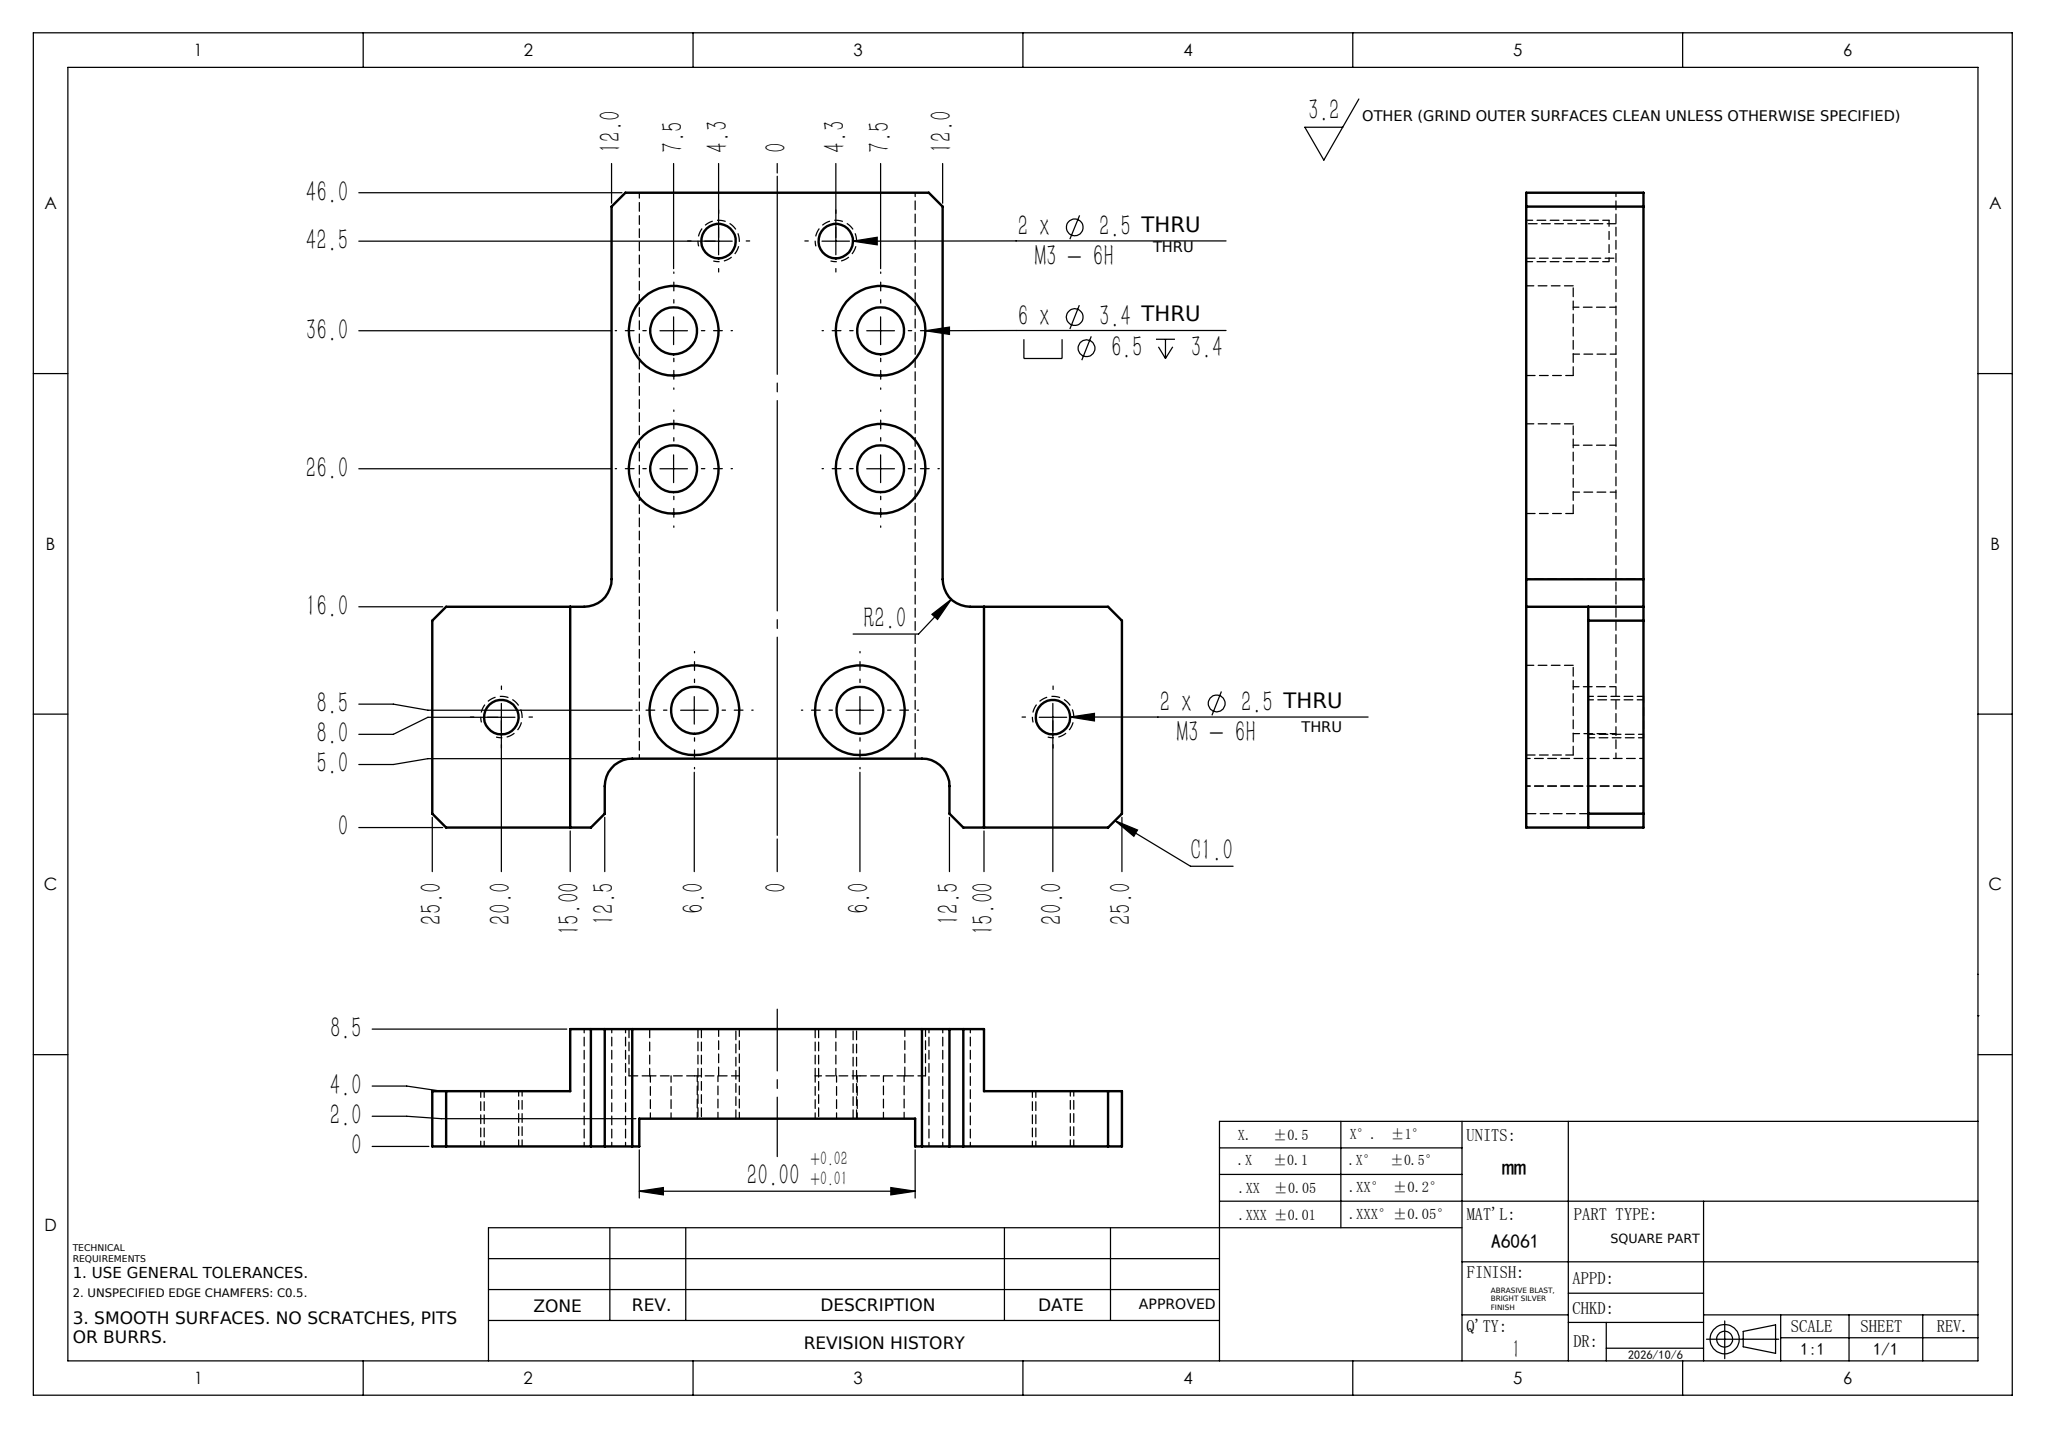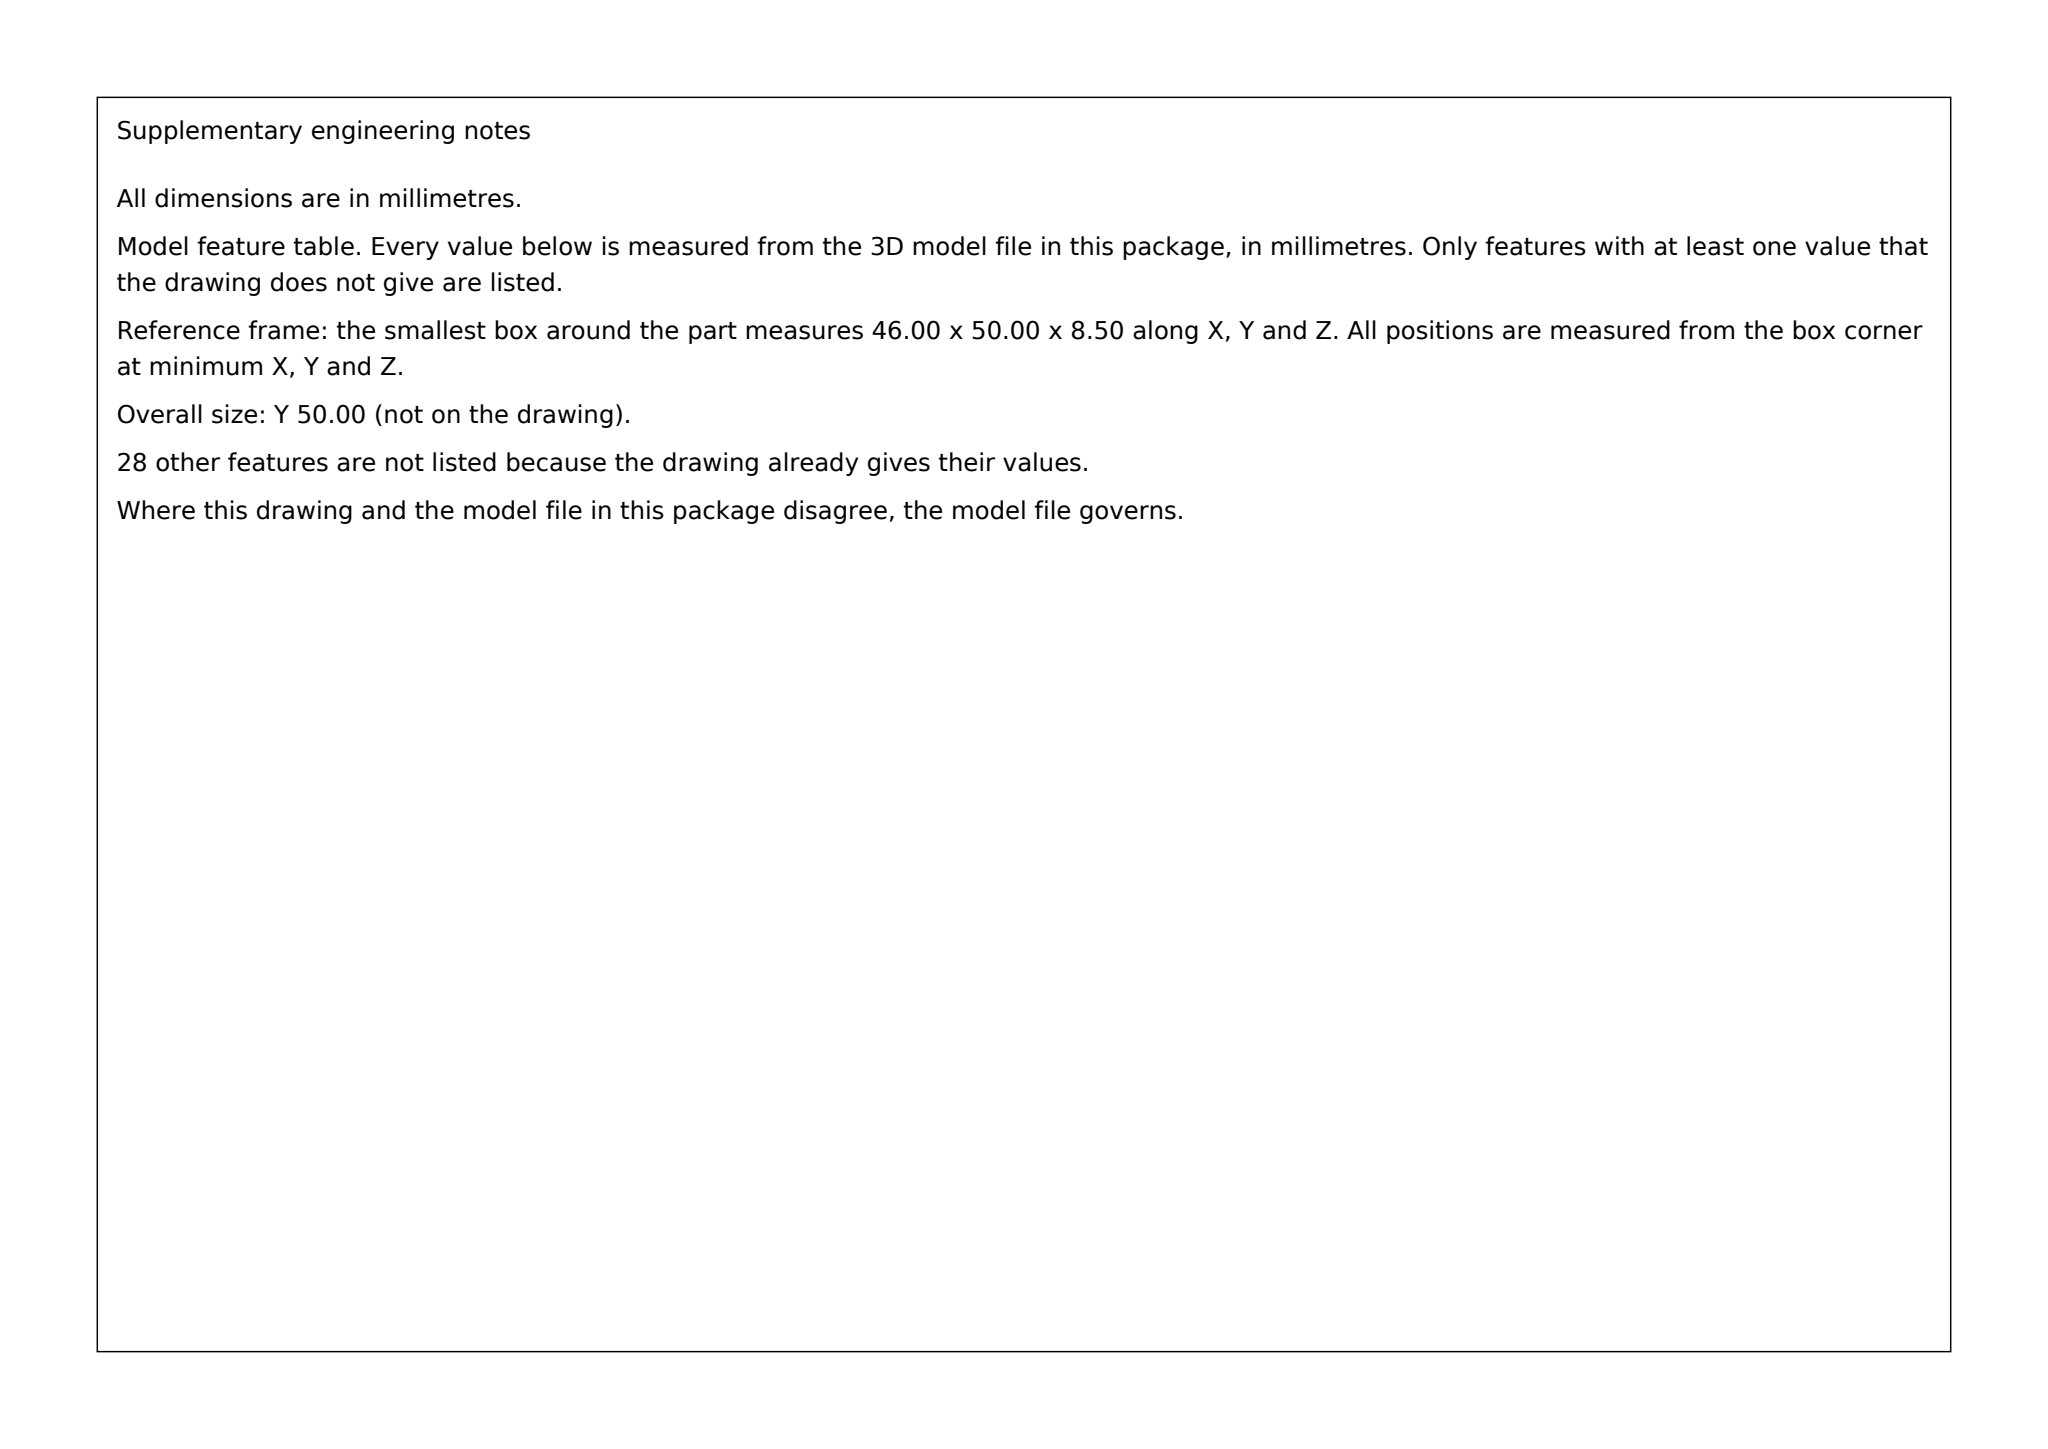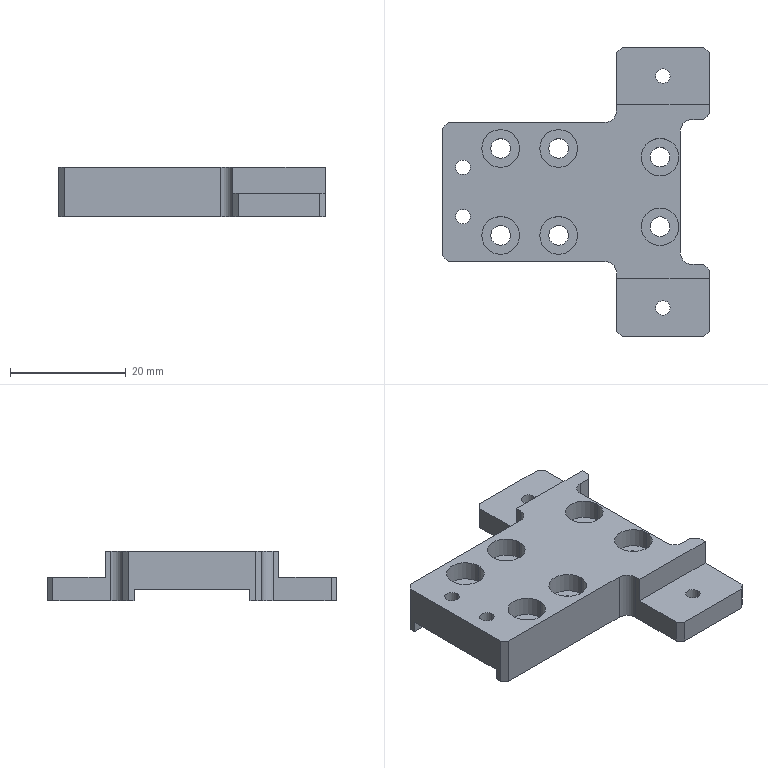Part | SolidWorks | mm | 1 solid | 72 faces | box 46 x 50 x 8.5 mm | volume 7833 mm3 | cylinder 36 | plane 36 | commonest cylinder face diameters 6.5 x12 3.4 x12 2.5 x8 4 x4
build123d program:
from build123d import *

# Parameters (mm, degrees)
SKETCH1_W                                       = 46
SKETCH1_H                                       = 50
BOSS_EXTRUDE1_DEPTH                             = 8.5
SKETCH2_W                                       = 30
SKETCH2_H                                       = 13
CUT_EXTRUDE1_DEPTH                              = 54.04
SKETCH3_W                                       = 46
SKETCH3_H                                       = 20
CUT_EXTRUDE2_DEPTH                              = 2
M3_HEX_SOCKET_HEAD_CAP_SCREW_CBORE1_D           = 3.4
M3_HEX_SOCKET_HEAD_CAP_SCREW_CBORE1_CBORE_D     = 6.5
M3_HEX_SOCKET_HEAD_CAP_SCREW_CBORE1_CBORE_DEPTH = 3.4
M3_TAPPED_HOLE1_D                               = 2.5
SKETCH9_W                                       = 16
SKETCH9_H                                       = 10
CUT_EXTRUDE3_DEPTH                              = 4.5
SKETCH11_W                                      = 5
SKETCH11_H                                      = 25
CUT_EXTRUDE4_DEPTH                              = 54.04
M3_TAPPED_HOLE2_D                               = 2.5
CHAMFER1_SIZE                                   = 1
FILLET1_R                                       = 2


with BuildPart() as part:
    # Sketch1 → Boss-Extrude1 (new body)
    with BuildSketch(Plane.XY):
        with Locations((23, 0)):
            Rectangle(SKETCH1_W, SKETCH1_H)
    extrude(amount=BOSS_EXTRUDE1_DEPTH)

    # Sketch2 → Cut-Extrude1 (cut, through all)
    with BuildSketch(Plane.XY.offset(8.5)):
        with Locations((15, 18.5)):
            Rectangle(SKETCH2_W, SKETCH2_H)
        with Locations((15, -18.5)):
            Rectangle(SKETCH2_W, SKETCH2_H)
    extrude(amount=-CUT_EXTRUDE1_DEPTH, mode=Mode.SUBTRACT)

    # Sketch3 → Cut-Extrude2 (cut)
    with BuildSketch(Plane(origin=(0, 0, 0), x_dir=(-1, 0, 0), z_dir=(0, 0, -1))):
        with Locations((-23, 0)):
            Rectangle(SKETCH3_W, SKETCH3_H)
    extrude(amount=-CUT_EXTRUDE2_DEPTH, mode=Mode.SUBTRACT)

    # M3 Hex Socket Head Cap Screw CBORE1 (through all)
    with Locations(Plane.XY.offset(8.5)):
        with Locations((10, -7.5), (10, 7.5), (20, 7.5), (20, -7.5), (37.5, -6), (37.5, 6)):
            CounterBoreHole(M3_HEX_SOCKET_HEAD_CAP_SCREW_CBORE1_D / 2, M3_HEX_SOCKET_HEAD_CAP_SCREW_CBORE1_CBORE_D / 2, M3_HEX_SOCKET_HEAD_CAP_SCREW_CBORE1_CBORE_DEPTH)

    # M3 Tapped Hole1 (through all)
    with Locations(Plane.XY.offset(8.5)):
        with Locations((3.5, -4.25), (3.5, 4.25)):
            Hole(M3_TAPPED_HOLE1_D / 2)

    # Sketch9 → Cut-Extrude3 (cut)
    with BuildSketch(Plane.XY.offset(8.5)):
        with Locations((38, -20)):
            Rectangle(SKETCH9_W, SKETCH9_H)
        with Locations((38, 20)):
            Rectangle(SKETCH9_W, SKETCH9_H)
    extrude(amount=-CUT_EXTRUDE3_DEPTH, mode=Mode.SUBTRACT)

    # Sketch11 → Cut-Extrude4 (cut, through all)
    with BuildSketch(Plane.XY.offset(8.5)):
        with Locations((43.5, 0)):
            Rectangle(SKETCH11_W, SKETCH11_H)
    extrude(amount=-CUT_EXTRUDE4_DEPTH, mode=Mode.SUBTRACT)

    # M3 Tapped Hole2 (through all)
    with Locations(Plane.XY.offset(4)):
        with Locations((38, -20), (38, 20)):
            Hole(M3_TAPPED_HOLE2_D / 2)

    # Chamfer1
    chamfer1_edges = [part.edges().sort_by_distance(p)[0] for p in [
        (46, -25, 2),
        (46, 25, 2),
        (46, 12.5, 4.25),
        (46, -12.5, 4.25),
        (0, 12, 4.25),
        (30, 25, 2),
        (30, -25, 2),
        (0, -12, 4.25),
    ]]
    chamfer(chamfer1_edges, length=CHAMFER1_SIZE)

    # Fillet1
    fillet1_edges = [part.edges().sort_by_distance(p)[0] for p in [
        (41, -12.5, 4.25),
        (41, 12.5, 4.25),
        (30, 12, 4.25),
        (30, -12, 4.25),
    ]]
    fillet(fillet1_edges, radius=FILLET1_R)


solid = part.part